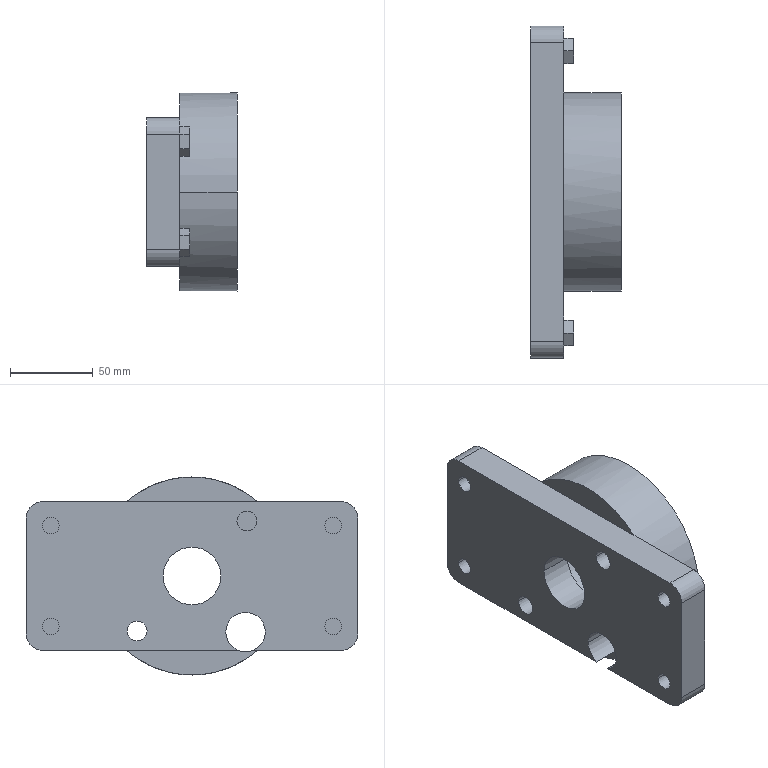Component | SolidWorks | FixedPlate-1 | 1 solid | 69 faces | box 55 x 201 x 120 mm | volume 574756 mm3 | plane 45 | cylinder 24 | commonest cylinder face diameters 10 x8 12 x4 20 x4 24 x2 35 x2 68 x2 120 x2
build123d program:
from build123d import *

# Parameters (mm, degrees)
SKETCH1_R           = 5
BOSS_EXTRUDE1_DEPTH = 20
SKETCH2_R           = 60
BOSS_EXTRUDE2_DEPTH = 35
SKETCH3_R           = 34
CUT_EXTRUDE1_DEPTH  = 35
SKETCH4_R           = 17.5
CUT_EXTRUDE2_DEPTH  = 35
SKETCH5_R           = 6
SKETCH5_R_2         = 12
CUT_EXTRUDE3_DEPTH  = 35
SKETCH6_R           = 6
CUT_EXTRUDE4_DEPTH  = 130.326
SKETCH7_R           = 6
SKETCH7_R_2         = 12
CUT_EXTRUDE5_DEPTH  = 130.326
SKETCH8_R           = 12
SKETCH8_R_2         = 6
BOSS_EXTRUDE3_DEPTH = 35
BOSS_EXTRUDE4_DEPTH = 6


with BuildPart() as part:
    # Sketch1 → Boss-Extrude1 (new body)
    with BuildSketch(Plane(origin=(0, 0, 0), x_dir=(0, 0, -1), z_dir=(1, 0, 0))):
        with BuildLine():
            Line((90.5, 45), (-90.5, 45))
            ThreePointArc((-90.5, 45), (-97.571, 42.071), (-100.5, 35))
            Line((-100.5, 35), (-100.5, -35))
            ThreePointArc((-100.5, -35), (-97.571, -42.071), (-90.5, -45))
            Line((-90.5, -45), (90.5, -45))
            ThreePointArc((90.5, -45), (97.571, -42.071), (100.5, -35))
            Line((100.5, -35), (100.5, 35))
            ThreePointArc((100.5, 35), (97.571, 42.071), (90.5, 45))
        make_face()
        with Locations((-85.5, 30.5)):
            Circle(SKETCH1_R, mode=Mode.SUBTRACT)
        with Locations((85.5, 30.5)):
            Circle(SKETCH1_R, mode=Mode.SUBTRACT)
        with Locations((-85.5, -30.5)):
            Circle(SKETCH1_R, mode=Mode.SUBTRACT)
        with Locations((85.5, -30.5)):
            Circle(SKETCH1_R, mode=Mode.SUBTRACT)
    extrude(amount=BOSS_EXTRUDE1_DEPTH)

    # Sketch2 → Boss-Extrude2 (add)
    with BuildSketch(Plane(origin=(20, 0, 0), x_dir=(0, 0, -1), z_dir=(1, 0, 0))):
        with Locations(Location((0, 0, 0), (0, 0, 131.41))):
            Circle(SKETCH2_R)
    extrude(amount=BOSS_EXTRUDE2_DEPTH)

    # Sketch3 → Cut-Extrude1 (cut)
    with BuildSketch(Plane(origin=(55, 0, 0), x_dir=(0, 0, -1), z_dir=(1, 0, 0))):
        Circle(SKETCH3_R)
    extrude(amount=-CUT_EXTRUDE1_DEPTH, mode=Mode.SUBTRACT)

    # Sketch4 → Cut-Extrude2 (cut)
    with BuildSketch(Plane.ZY):
        Circle(SKETCH4_R)
    extrude(amount=-CUT_EXTRUDE2_DEPTH, mode=Mode.SUBTRACT)

    # Sketch5 → Cut-Extrude3 (cut)
    with BuildSketch(Plane(origin=(55, 0, 0), x_dir=(0, 0, -1), z_dir=(1, 0, 0))):
        with Locations((33.234, -33.234)):
            Circle(SKETCH5_R)
        with Locations((-32.45, -34)):
            Circle(SKETCH5_R_2)
    extrude(amount=-CUT_EXTRUDE3_DEPTH, mode=Mode.SUBTRACT)

    # Sketch6 → Cut-Extrude4 (cut, through all)
    with BuildSketch(Plane(origin=(55, 0, 0), x_dir=(0, 0, -1), z_dir=(1, 0, 0))):
        with Locations((33.234, -33.234)):
            Circle(SKETCH6_R)
    extrude(amount=-CUT_EXTRUDE4_DEPTH, mode=Mode.SUBTRACT)

    # Sketch7 → Cut-Extrude5 (cut, through all)
    with BuildSketch(Plane(origin=(55, 0, 0), x_dir=(0, 0, -1), z_dir=(1, 0, 0))):
        with Locations((-33.234, 33.234)):
            Circle(SKETCH7_R)
        with Locations((32.45, 34)):
            Circle(SKETCH7_R_2)
    extrude(amount=-CUT_EXTRUDE5_DEPTH, mode=Mode.SUBTRACT)

    # Sketch8 → Boss-Extrude3 (add)
    with BuildSketch(Plane(origin=(55, 0, 0), x_dir=(0, 0, -1), z_dir=(1, 0, 0))):
        with Locations((-32.45, -34)):
            Circle(SKETCH8_R)
        with Locations((33.234, -33.234)):
            Circle(SKETCH8_R_2)
    extrude(amount=-BOSS_EXTRUDE3_DEPTH)

    # Sketch9 → Boss-Extrude4 (add)
    with BuildSketch(Plane(origin=(20, 0, 0), x_dir=(0, 0, -1), z_dir=(1, 0, 0))):
        Polygon((-85.5, 22.036), (-78.17, 26.268), (-78.17, 34.732), (-85.5, 38.964), (-92.83, 34.732), (-92.83, 26.268), align=None)
        Polygon((-85.5, -39.397), (-77.795, -34.949), (-77.795, -26.051), (-85.5, -21.603), (-93.205, -26.051), (-93.205, -34.949), align=None)
        Polygon((85.5, 22.036), (92.83, 26.268), (92.83, 34.732), (85.5, 38.964), (78.17, 34.732), (78.17, 26.268), align=None)
        Polygon((85.5, -39.397), (93.205, -34.949), (93.205, -26.051), (85.5, -21.603), (77.795, -26.051), (77.795, -34.949), align=None)
    extrude(amount=BOSS_EXTRUDE4_DEPTH)


solid = part.part

# Placed as in the assembly
solid = solid.moved(Location((439.733, 15.31, -240), (-90, 0, 0)))